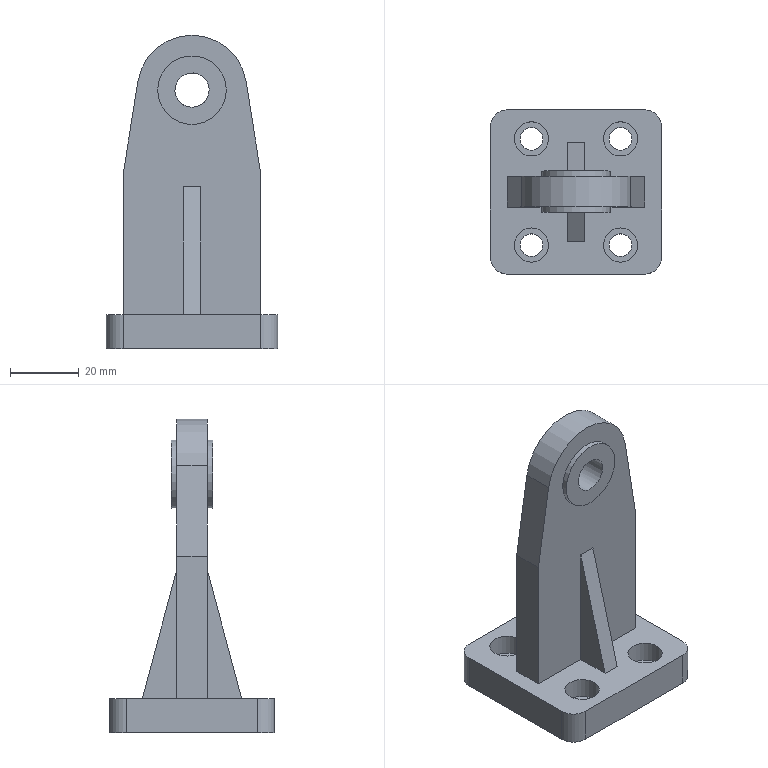Component | NX | BRACKET_B | 1 solid | 40 faces | volume 49600 mm3 | plane 24 | cylinder 16 | commonest cylinder face diameters 10 x9 6.6 x4 20 x2 32 x1